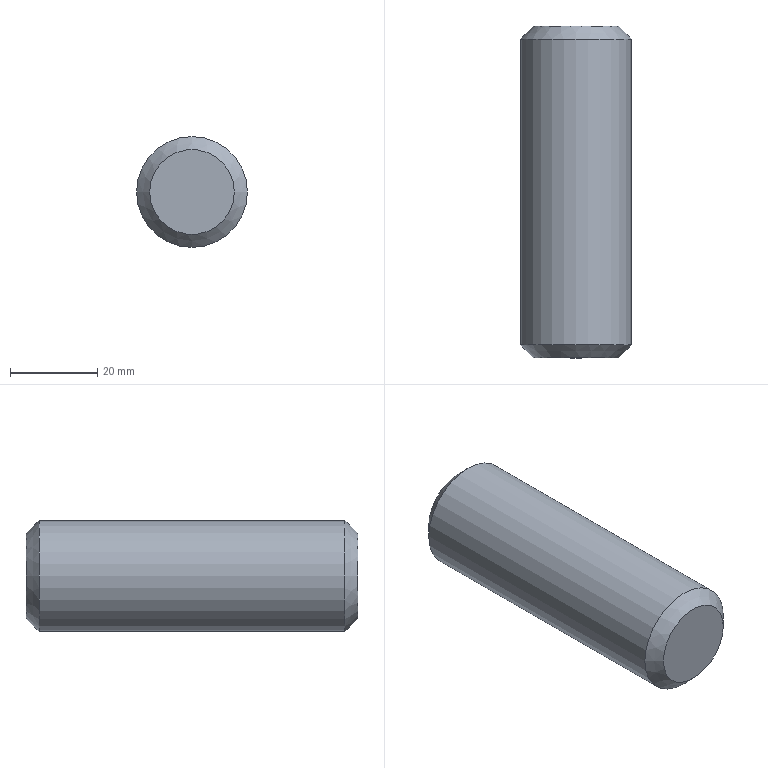Component | NX | PIN_76 | 1 solid | 5 faces | volume 37848 mm3 | plane 2 | cone 2 | cylinder 1 | commonest cylinder face diameters 25.4 x1